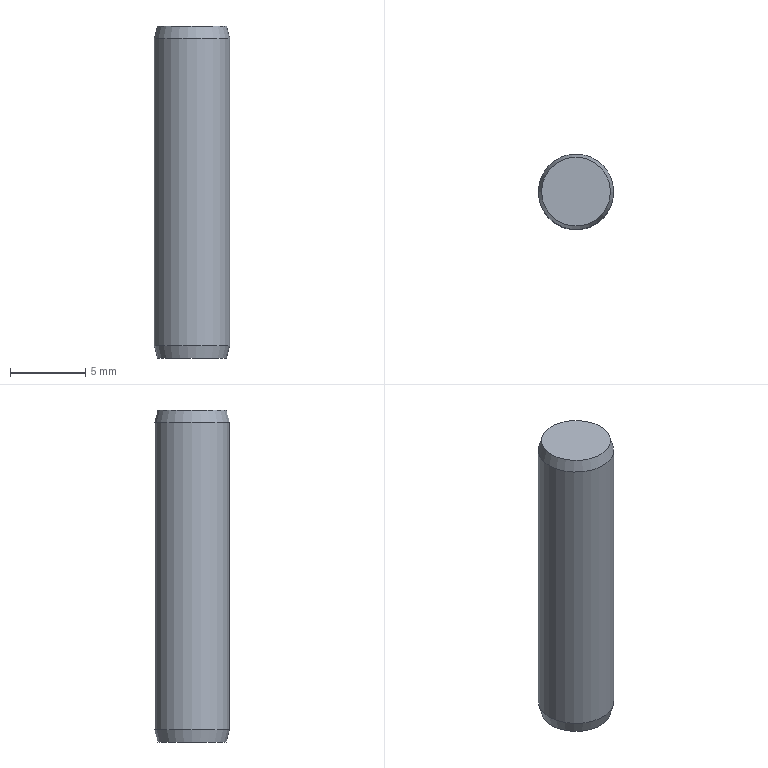Component | NX | GB-T119_1-2000_5X22 | 1 solid | 5 faces | box 5 x 5 x 22 mm | volume 429 mm3 | plane 2 | cone 2 | cylinder 1 | commonest cylinder face diameters 5 x1
STEP:
#1=CARTESIAN_POINT('',(0.,0.,0.));
#2=DIRECTION('',(0.,0.,1.));
#3=DIRECTION('',(1.,0.,0.));
#4=AXIS2_PLACEMENT_3D('',#1,#2,#3);
#5=CARTESIAN_POINT('',(-39.286,-12.5,-27.));
#6=VERTEX_POINT('',#5);
#7=CARTESIAN_POINT('',(-37.,-12.5,-27.));
#8=DIRECTION('',(0.,0.,-1.));
#9=DIRECTION('',(-1.,0.,0.));
#10=AXIS2_PLACEMENT_3D('',#7,#8,#9);
#11=CIRCLE('',#10,2.286);
#12=CARTESIAN_POINT('',(-37.,-12.5,-27.));
#13=DIRECTION('',(0.,0.,-1.));
#14=DIRECTION('',(-1.,0.,0.));
#15=AXIS2_PLACEMENT_3D('',#12,#13,#14);
#16=PLANE('',#15);
#17=CARTESIAN_POINT('',(0.,0.));
#18=DIRECTION('',(1.,0.));
#19=AXIS2_PLACEMENT_2D('',#17,#18);
#20=CIRCLE('',#19,2.286);
#21=(GEOMETRIC_REPRESENTATION_CONTEXT(2)PARAMETRIC_REPRESENTATION_CONTEXT()REPRESENTATION_CONTEXT('',''));
#22=DEFINITIONAL_REPRESENTATION('',(#20),#21);
#23=PCURVE('',#16,#22);
#24=CARTESIAN_POINT('',(-37.,-12.5,-27.));
#25=DIRECTION('',(0.,0.,1.));
#26=DIRECTION('',(1.,0.,0.));
#27=AXIS2_PLACEMENT_3D('',#24,#25,#26);
#28=CONICAL_SURFACE('',#27,2.286,0.2618);
#29=CARTESIAN_POINT('',(9.425,-0.));
#30=DIRECTION('',(-1.,0.));
#31=VECTOR('',#30,1.);
#32=LINE('',#29,#31);
#33=(GEOMETRIC_REPRESENTATION_CONTEXT(2)PARAMETRIC_REPRESENTATION_CONTEXT()REPRESENTATION_CONTEXT('',''));
#34=DEFINITIONAL_REPRESENTATION('',(#32),#33);
#35=PCURVE('',#28,#34);
#36=SURFACE_CURVE('',#11,(#23,#35),.PCURVE_S1.);
#37=EDGE_CURVE('',#6,#6,#36,.T.);
#38=ORIENTED_EDGE('',*,*,#37,.T.);
#39=EDGE_LOOP('',(#38));
#40=FACE_BOUND('',#39,.T.);
#41=ADVANCED_FACE('',(#40),#16,.T.);
#42=CARTESIAN_POINT('',(-39.5,-12.5,-26.2));
#43=VERTEX_POINT('',#42);
#44=CARTESIAN_POINT('',(-37.,-12.5,-26.2));
#45=DIRECTION('',(0.,0.,-1.));
#46=DIRECTION('',(-1.,0.,0.));
#47=AXIS2_PLACEMENT_3D('',#44,#45,#46);
#48=CIRCLE('',#47,2.5);
#49=CARTESIAN_POINT('',(9.425,0.8));
#50=DIRECTION('',(-1.,0.));
#51=VECTOR('',#50,1.);
#52=LINE('',#49,#51);
#53=(GEOMETRIC_REPRESENTATION_CONTEXT(2)PARAMETRIC_REPRESENTATION_CONTEXT()REPRESENTATION_CONTEXT('',''));
#54=DEFINITIONAL_REPRESENTATION('',(#52),#53);
#55=PCURVE('',#28,#54);
#56=CARTESIAN_POINT('',(-37.,-12.5,-5.));
#57=DIRECTION('',(0.,0.,-1.));
#58=DIRECTION('',(-1.,0.,0.));
#59=AXIS2_PLACEMENT_3D('',#56,#57,#58);
#60=CYLINDRICAL_SURFACE('',#59,2.5);
#61=CARTESIAN_POINT('',(0.,21.2));
#62=DIRECTION('',(1.,0.));
#63=VECTOR('',#62,1.);
#64=LINE('',#61,#63);
#65=(GEOMETRIC_REPRESENTATION_CONTEXT(2)PARAMETRIC_REPRESENTATION_CONTEXT()REPRESENTATION_CONTEXT('',''));
#66=DEFINITIONAL_REPRESENTATION('',(#64),#65);
#67=PCURVE('',#60,#66);
#68=SURFACE_CURVE('',#48,(#55,#67),.PCURVE_S1.);
#69=EDGE_CURVE('',#43,#43,#68,.T.);
#70=ORIENTED_EDGE('',*,*,#69,.T.);
#71=CARTESIAN_POINT('',(-39.286,-12.5,-27.));
#72=CARTESIAN_POINT('',(-39.5,-12.5,-26.2));
#73=B_SPLINE_CURVE_WITH_KNOTS('',1,(#71,#72),.UNSPECIFIED.,.F.,.F.,(2,2),(-0.,0.8282),.PIECEWISE_BEZIER_KNOTS.);
#74=CARTESIAN_POINT('',(3.142,0.));
#75=DIRECTION('',(0.,1.));
#76=VECTOR('',#75,1.);
#77=LINE('',#74,#76);
#78=(GEOMETRIC_REPRESENTATION_CONTEXT(2)PARAMETRIC_REPRESENTATION_CONTEXT()REPRESENTATION_CONTEXT('',''));
#79=DEFINITIONAL_REPRESENTATION('',(#77),#78);
#80=PCURVE('',#28,#79);
#81=CARTESIAN_POINT('',(9.425,0.));
#82=DIRECTION('',(0.,1.));
#83=VECTOR('',#82,1.);
#84=LINE('',#81,#83);
#85=(GEOMETRIC_REPRESENTATION_CONTEXT(2)PARAMETRIC_REPRESENTATION_CONTEXT()REPRESENTATION_CONTEXT('',''));
#86=DEFINITIONAL_REPRESENTATION('',(#84),#85);
#87=PCURVE('',#28,#86);
#88=SEAM_CURVE('',#73,(#80,#87),.PCURVE_S1.);
#89=EDGE_CURVE('',#6,#43,#88,.T.);
#90=ORIENTED_EDGE('',*,*,#89,.F.);
#91=ORIENTED_EDGE('',*,*,#37,.F.);
#92=ORIENTED_EDGE('',*,*,#89,.T.);
#93=EDGE_LOOP('',(#70,#90,#91,#92));
#94=FACE_BOUND('',#93,.T.);
#95=ADVANCED_FACE('',(#94),#28,.T.);
#96=CARTESIAN_POINT('',(-39.5,-12.5,-5.8));
#97=VERTEX_POINT('',#96);
#98=CARTESIAN_POINT('',(-37.,-12.5,-5.8));
#99=DIRECTION('',(0.,0.,-1.));
#100=DIRECTION('',(-1.,0.,0.));
#101=AXIS2_PLACEMENT_3D('',#98,#99,#100);
#102=CIRCLE('',#101,2.5);
#103=CARTESIAN_POINT('',(0.,0.8));
#104=DIRECTION('',(1.,0.));
#105=VECTOR('',#104,1.);
#106=LINE('',#103,#105);
#107=(GEOMETRIC_REPRESENTATION_CONTEXT(2)PARAMETRIC_REPRESENTATION_CONTEXT()REPRESENTATION_CONTEXT('',''));
#108=DEFINITIONAL_REPRESENTATION('',(#106),#107);
#109=PCURVE('',#60,#108);
#110=CARTESIAN_POINT('',(-37.,-12.5,-5.8));
#111=DIRECTION('',(0.,0.,-1.));
#112=DIRECTION('',(-1.,0.,0.));
#113=AXIS2_PLACEMENT_3D('',#110,#111,#112);
#114=CONICAL_SURFACE('',#113,2.5,0.2618);
#115=CARTESIAN_POINT('',(0.,-0.));
#116=DIRECTION('',(1.,0.));
#117=VECTOR('',#116,1.);
#118=LINE('',#115,#117);
#119=(GEOMETRIC_REPRESENTATION_CONTEXT(2)PARAMETRIC_REPRESENTATION_CONTEXT()REPRESENTATION_CONTEXT('',''));
#120=DEFINITIONAL_REPRESENTATION('',(#118),#119);
#121=PCURVE('',#114,#120);
#122=SURFACE_CURVE('',#102,(#109,#121),.PCURVE_S1.);
#123=EDGE_CURVE('',#97,#97,#122,.T.);
#124=ORIENTED_EDGE('',*,*,#123,.T.);
#125=CARTESIAN_POINT('',(-39.5,-12.5,-5.8));
#126=CARTESIAN_POINT('',(-39.5,-12.5,-26.2));
#127=B_SPLINE_CURVE_WITH_KNOTS('',1,(#125,#126),.UNSPECIFIED.,.F.,.F.,(2,2),(0.8,21.2),.PIECEWISE_BEZIER_KNOTS.);
#128=CARTESIAN_POINT('',(6.283,0.));
#129=DIRECTION('',(0.,1.));
#130=VECTOR('',#129,1.);
#131=LINE('',#128,#130);
#132=(GEOMETRIC_REPRESENTATION_CONTEXT(2)PARAMETRIC_REPRESENTATION_CONTEXT()REPRESENTATION_CONTEXT('',''));
#133=DEFINITIONAL_REPRESENTATION('',(#131),#132);
#134=PCURVE('',#60,#133);
#135=CARTESIAN_POINT('',(0.,0.));
#136=DIRECTION('',(0.,1.));
#137=VECTOR('',#136,1.);
#138=LINE('',#135,#137);
#139=(GEOMETRIC_REPRESENTATION_CONTEXT(2)PARAMETRIC_REPRESENTATION_CONTEXT()REPRESENTATION_CONTEXT('',''));
#140=DEFINITIONAL_REPRESENTATION('',(#138),#139);
#141=PCURVE('',#60,#140);
#142=SEAM_CURVE('',#127,(#134,#141),.PCURVE_S1.);
#143=EDGE_CURVE('',#97,#43,#142,.T.);
#144=ORIENTED_EDGE('',*,*,#143,.T.);
#145=ORIENTED_EDGE('',*,*,#69,.F.);
#146=ORIENTED_EDGE('',*,*,#143,.F.);
#147=EDGE_LOOP('',(#124,#144,#145,#146));
#148=FACE_BOUND('',#147,.T.);
#149=ADVANCED_FACE('',(#148),#60,.T.);
#150=CARTESIAN_POINT('',(-39.286,-12.5,-5.));
#151=VERTEX_POINT('',#150);
#152=CARTESIAN_POINT('',(-37.,-12.5,-5.));
#153=DIRECTION('',(0.,0.,-1.));
#154=DIRECTION('',(-1.,0.,0.));
#155=AXIS2_PLACEMENT_3D('',#152,#153,#154);
#156=CIRCLE('',#155,2.286);
#157=CARTESIAN_POINT('',(0.,-0.8));
#158=DIRECTION('',(1.,0.));
#159=VECTOR('',#158,1.);
#160=LINE('',#157,#159);
#161=(GEOMETRIC_REPRESENTATION_CONTEXT(2)PARAMETRIC_REPRESENTATION_CONTEXT()REPRESENTATION_CONTEXT('',''));
#162=DEFINITIONAL_REPRESENTATION('',(#160),#161);
#163=PCURVE('',#114,#162);
#164=CARTESIAN_POINT('',(-34.714,-12.5,-5.));
#165=DIRECTION('',(0.,0.,1.));
#166=DIRECTION('',(1.,0.,0.));
#167=AXIS2_PLACEMENT_3D('',#164,#165,#166);
#168=PLANE('',#167);
#169=CARTESIAN_POINT('',(-4.571,0.));
#170=CARTESIAN_POINT('',(-4.571,3.959));
#171=CARTESIAN_POINT('',(-1.143,1.979));
#172=CARTESIAN_POINT('',(2.286,0.));
#173=CARTESIAN_POINT('',(-1.143,-1.979));
#174=CARTESIAN_POINT('',(-4.571,-3.959));
#175=CARTESIAN_POINT('',(-4.571,0.));
#176=(BOUNDED_CURVE()B_SPLINE_CURVE(2,(#169,#170,#171,#172,#173,#174,#175),.UNSPECIFIED.,.T.,.F.)B_SPLINE_CURVE_WITH_KNOTS((1,2,2,2,2,1),(-2.094,0.,2.094,4.189,6.283,8.378),.UNSPECIFIED.)CURVE()GEOMETRIC_REPRESENTATION_ITEM()RATIONAL_B_SPLINE_CURVE((1.,0.5,1.,0.5,1.,0.5,1.))REPRESENTATION_ITEM(''));
#177=(GEOMETRIC_REPRESENTATION_CONTEXT(2)PARAMETRIC_REPRESENTATION_CONTEXT()REPRESENTATION_CONTEXT('',''));
#178=DEFINITIONAL_REPRESENTATION('',(#176),#177);
#179=PCURVE('',#168,#178);
#180=SURFACE_CURVE('',#156,(#163,#179),.PCURVE_S1.);
#181=EDGE_CURVE('',#151,#151,#180,.T.);
#182=ORIENTED_EDGE('',*,*,#181,.T.);
#183=CARTESIAN_POINT('',(-39.286,-12.5,-5.));
#184=CARTESIAN_POINT('',(-39.5,-12.5,-5.8));
#185=B_SPLINE_CURVE_WITH_KNOTS('',1,(#183,#184),.UNSPECIFIED.,.F.,.F.,(2,2),(-0.8282,-0.),.PIECEWISE_BEZIER_KNOTS.);
#186=CARTESIAN_POINT('',(6.283,0.));
#187=DIRECTION('',(0.,1.));
#188=VECTOR('',#187,1.);
#189=LINE('',#186,#188);
#190=(GEOMETRIC_REPRESENTATION_CONTEXT(2)PARAMETRIC_REPRESENTATION_CONTEXT()REPRESENTATION_CONTEXT('',''));
#191=DEFINITIONAL_REPRESENTATION('',(#189),#190);
#192=PCURVE('',#114,#191);
#193=CARTESIAN_POINT('',(0.,0.));
#194=DIRECTION('',(0.,1.));
#195=VECTOR('',#194,1.);
#196=LINE('',#193,#195);
#197=(GEOMETRIC_REPRESENTATION_CONTEXT(2)PARAMETRIC_REPRESENTATION_CONTEXT()REPRESENTATION_CONTEXT('',''));
#198=DEFINITIONAL_REPRESENTATION('',(#196),#197);
#199=PCURVE('',#114,#198);
#200=SEAM_CURVE('',#185,(#192,#199),.PCURVE_S1.);
#201=EDGE_CURVE('',#151,#97,#200,.T.);
#202=ORIENTED_EDGE('',*,*,#201,.T.);
#203=ORIENTED_EDGE('',*,*,#123,.F.);
#204=ORIENTED_EDGE('',*,*,#201,.F.);
#205=EDGE_LOOP('',(#182,#202,#203,#204));
#206=FACE_BOUND('',#205,.T.);
#207=ADVANCED_FACE('',(#206),#114,.T.);
#208=ORIENTED_EDGE('',*,*,#181,.F.);
#209=EDGE_LOOP('',(#208));
#210=FACE_BOUND('',#209,.T.);
#211=ADVANCED_FACE('',(#210),#168,.T.);
#212=CLOSED_SHELL('',(#41,#95,#149,#207,#211));
#213=MANIFOLD_SOLID_BREP('',#212);
#214=(LENGTH_UNIT()NAMED_UNIT(*)SI_UNIT(.MILLI.,.METRE.));
#215=UNCERTAINTY_MEASURE_WITH_UNIT(LENGTH_MEASURE(0.00001),#214,'','');
#216=(NAMED_UNIT(*)PLANE_ANGLE_UNIT()SI_UNIT($,.RADIAN.));
#217=(NAMED_UNIT(*)SI_UNIT($,.STERADIAN.)SOLID_ANGLE_UNIT());
#218=(GEOMETRIC_REPRESENTATION_CONTEXT(3)GLOBAL_UNCERTAINTY_ASSIGNED_CONTEXT((#215))GLOBAL_UNIT_ASSIGNED_CONTEXT((#214,#216,#217))REPRESENTATION_CONTEXT('',''));
#219=ADVANCED_BREP_SHAPE_REPRESENTATION('',(#4,#213),#218);